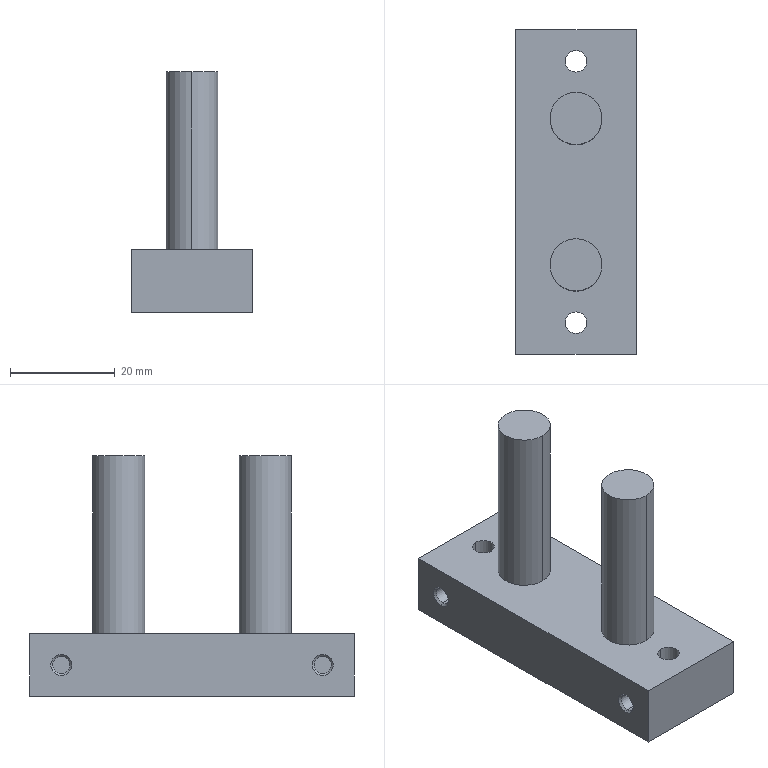Component | SolidWorks | P-SLJ-005-3_CXSM20-20-Z73-1_rod CXSM20-20-Z73-1 | 1 solid | 40 faces | box 23 x 62 x 46 mm | volume 21928 mm3 | cylinder 16 | cone 12 | plane 12 | commonest cylinder face diameters 3.24 x8 4.13 x4 10 x4
STEP:
#1=COLOUR_RGB('',0.7922,0.8196,0.9333);
#2=FILL_AREA_STYLE_COLOUR('',#1);
#3=FILL_AREA_STYLE('',(#2));
#4=SURFACE_STYLE_FILL_AREA(#3);
#5=SURFACE_SIDE_STYLE('',(#4));
#6=SURFACE_STYLE_USAGE(.BOTH.,#5);
#7=PRESENTATION_STYLE_ASSIGNMENT((#6));
#8=CARTESIAN_POINT('',(-2.003,1.594,49.262));
#9=VERTEX_POINT('',#8);
#10=CARTESIAN_POINT('',(-2.003,1.594,49.134));
#11=VERTEX_POINT('',#10);
#12=CARTESIAN_POINT('',(-2.003,1.594,49.198));
#13=DIRECTION('',(-1.,-0.,-0.));
#14=DIRECTION('',(0.,0.,-1.));
#15=AXIS2_PLACEMENT_3D('',#12,#13,#14);
#16=CIRCLE('',#15,0.06378);
#17=EDGE_CURVE('',#9,#11,#16,.T.);
#18=ORIENTED_EDGE('',*,*,#17,.F.);
#19=CARTESIAN_POINT('',(-2.224,1.594,49.262));
#20=VERTEX_POINT('',#19);
#21=CARTESIAN_POINT('',(-1.949,1.594,49.262));
#22=DIRECTION('',(-1.,-0.,-0.));
#23=VECTOR('',#22,39.37);
#24=LINE('',#21,#23);
#25=EDGE_CURVE('',#9,#20,#24,.T.);
#26=ORIENTED_EDGE('',*,*,#25,.T.);
#27=CARTESIAN_POINT('',(-2.224,1.594,49.134));
#28=VERTEX_POINT('',#27);
#29=CARTESIAN_POINT('',(-2.224,1.594,49.198));
#30=DIRECTION('',(-1.,-0.,-0.));
#31=DIRECTION('',(0.,0.,-1.));
#32=AXIS2_PLACEMENT_3D('',#29,#30,#31);
#33=CIRCLE('',#32,0.06378);
#34=EDGE_CURVE('',#20,#28,#33,.T.);
#35=ORIENTED_EDGE('',*,*,#34,.T.);
#36=CARTESIAN_POINT('',(-1.949,1.594,49.134));
#37=DIRECTION('',(-1.,-0.,-0.));
#38=VECTOR('',#37,39.37);
#39=LINE('',#36,#38);
#40=EDGE_CURVE('',#11,#28,#39,.T.);
#41=ORIENTED_EDGE('',*,*,#40,.F.);
#42=EDGE_LOOP('',(#18,#26,#35,#41));
#43=FACE_OUTER_BOUND('',#42,.T.);
#44=CARTESIAN_POINT('',(-1.949,1.594,49.198));
#45=DIRECTION('',(-1.,-0.,-0.));
#46=DIRECTION('',(0.,0.,-1.));
#47=AXIS2_PLACEMENT_3D('',#44,#45,#46);
#48=CYLINDRICAL_SURFACE('',#47,0.06378);
#49=ADVANCED_FACE('',(#43),#48,.F.);
#50=ORIENTED_EDGE('',*,*,#17,.T.);
#51=CARTESIAN_POINT('',(-1.988,1.594,49.119));
#52=VERTEX_POINT('',#51);
#53=CARTESIAN_POINT('',(-1.949,1.594,49.08));
#54=DIRECTION('',(0.7071,0.,-0.7071));
#55=VECTOR('',#54,39.37);
#56=LINE('',#53,#55);
#57=EDGE_CURVE('',#11,#52,#56,.T.);
#58=ORIENTED_EDGE('',*,*,#57,.T.);
#59=CARTESIAN_POINT('',(-1.988,1.594,49.277));
#60=VERTEX_POINT('',#59);
#61=CARTESIAN_POINT('',(-1.988,1.594,49.198));
#62=DIRECTION('',(1.,0.,0.));
#63=DIRECTION('',(0.,0.,-1.));
#64=AXIS2_PLACEMENT_3D('',#61,#62,#63);
#65=CIRCLE('',#64,0.07874);
#66=EDGE_CURVE('',#52,#60,#65,.T.);
#67=ORIENTED_EDGE('',*,*,#66,.T.);
#68=CARTESIAN_POINT('',(-1.949,1.594,49.316));
#69=DIRECTION('',(0.7071,0.,0.7071));
#70=VECTOR('',#69,39.37);
#71=LINE('',#68,#70);
#72=EDGE_CURVE('',#9,#60,#71,.T.);
#73=ORIENTED_EDGE('',*,*,#72,.F.);
#74=EDGE_LOOP('',(#50,#58,#67,#73));
#75=FACE_OUTER_BOUND('',#74,.T.);
#76=CARTESIAN_POINT('',(-1.949,1.594,49.198));
#77=DIRECTION('',(1.,0.,0.));
#78=DIRECTION('',(0.,0.,1.));
#79=AXIS2_PLACEMENT_3D('',#76,#77,#78);
#80=CONICAL_SURFACE('',#79,0.1181,0.7854);
#81=ADVANCED_FACE('',(#75),#80,.F.);
#82=CARTESIAN_POINT('',(-2.003,-0.374,49.262));
#83=VERTEX_POINT('',#82);
#84=CARTESIAN_POINT('',(-2.003,-0.374,49.134));
#85=VERTEX_POINT('',#84);
#86=CARTESIAN_POINT('',(-2.003,-0.374,49.198));
#87=DIRECTION('',(-1.,-0.,-0.));
#88=DIRECTION('',(0.,0.,-1.));
#89=AXIS2_PLACEMENT_3D('',#86,#87,#88);
#90=CIRCLE('',#89,0.06378);
#91=EDGE_CURVE('',#83,#85,#90,.T.);
#92=ORIENTED_EDGE('',*,*,#91,.F.);
#93=CARTESIAN_POINT('',(-2.224,-0.374,49.262));
#94=VERTEX_POINT('',#93);
#95=CARTESIAN_POINT('',(-1.949,-0.374,49.262));
#96=DIRECTION('',(-1.,-0.,-0.));
#97=VECTOR('',#96,39.37);
#98=LINE('',#95,#97);
#99=EDGE_CURVE('',#83,#94,#98,.T.);
#100=ORIENTED_EDGE('',*,*,#99,.T.);
#101=CARTESIAN_POINT('',(-2.224,-0.374,49.134));
#102=VERTEX_POINT('',#101);
#103=CARTESIAN_POINT('',(-2.224,-0.374,49.198));
#104=DIRECTION('',(-1.,-0.,-0.));
#105=DIRECTION('',(0.,0.,-1.));
#106=AXIS2_PLACEMENT_3D('',#103,#104,#105);
#107=CIRCLE('',#106,0.06378);
#108=EDGE_CURVE('',#94,#102,#107,.T.);
#109=ORIENTED_EDGE('',*,*,#108,.T.);
#110=CARTESIAN_POINT('',(-1.949,-0.374,49.134));
#111=DIRECTION('',(-1.,-0.,-0.));
#112=VECTOR('',#111,39.37);
#113=LINE('',#110,#112);
#114=EDGE_CURVE('',#85,#102,#113,.T.);
#115=ORIENTED_EDGE('',*,*,#114,.F.);
#116=EDGE_LOOP('',(#92,#100,#109,#115));
#117=FACE_OUTER_BOUND('',#116,.T.);
#118=CARTESIAN_POINT('',(-1.949,-0.374,49.198));
#119=DIRECTION('',(-1.,-0.,-0.));
#120=DIRECTION('',(0.,0.,-1.));
#121=AXIS2_PLACEMENT_3D('',#118,#119,#120);
#122=CYLINDRICAL_SURFACE('',#121,0.06378);
#123=ADVANCED_FACE('',(#117),#122,.F.);
#124=ORIENTED_EDGE('',*,*,#91,.T.);
#125=CARTESIAN_POINT('',(-1.988,-0.374,49.119));
#126=VERTEX_POINT('',#125);
#127=CARTESIAN_POINT('',(-1.949,-0.374,49.08));
#128=DIRECTION('',(0.7071,0.,-0.7071));
#129=VECTOR('',#128,39.37);
#130=LINE('',#127,#129);
#131=EDGE_CURVE('',#85,#126,#130,.T.);
#132=ORIENTED_EDGE('',*,*,#131,.T.);
#133=CARTESIAN_POINT('',(-1.988,-0.374,49.277));
#134=VERTEX_POINT('',#133);
#135=CARTESIAN_POINT('',(-1.988,-0.374,49.198));
#136=DIRECTION('',(1.,0.,0.));
#137=DIRECTION('',(0.,0.,-1.));
#138=AXIS2_PLACEMENT_3D('',#135,#136,#137);
#139=CIRCLE('',#138,0.07874);
#140=EDGE_CURVE('',#126,#134,#139,.T.);
#141=ORIENTED_EDGE('',*,*,#140,.T.);
#142=CARTESIAN_POINT('',(-1.949,-0.374,49.316));
#143=DIRECTION('',(0.7071,0.,0.7071));
#144=VECTOR('',#143,39.37);
#145=LINE('',#142,#144);
#146=EDGE_CURVE('',#83,#134,#145,.T.);
#147=ORIENTED_EDGE('',*,*,#146,.F.);
#148=EDGE_LOOP('',(#124,#132,#141,#147));
#149=FACE_OUTER_BOUND('',#148,.T.);
#150=CARTESIAN_POINT('',(-1.949,-0.374,49.198));
#151=DIRECTION('',(1.,0.,0.));
#152=DIRECTION('',(0.,0.,1.));
#153=AXIS2_PLACEMENT_3D('',#150,#151,#152);
#154=CONICAL_SURFACE('',#153,0.1181,0.7854);
#155=ADVANCED_FACE('',(#149),#154,.F.);
#156=CARTESIAN_POINT('',(-2.441,1.513,48.979));
#157=VERTEX_POINT('',#156);
#158=CARTESIAN_POINT('',(-2.441,1.676,48.979));
#159=VERTEX_POINT('',#158);
#160=CARTESIAN_POINT('',(-2.441,1.594,48.979));
#161=DIRECTION('',(-0.,0.,1.));
#162=DIRECTION('',(0.,1.,0.));
#163=AXIS2_PLACEMENT_3D('',#160,#161,#162);
#164=CIRCLE('',#163,0.0813);
#165=EDGE_CURVE('',#157,#159,#164,.T.);
#166=ORIENTED_EDGE('',*,*,#165,.T.);
#167=CARTESIAN_POINT('',(-2.441,1.693,48.962));
#168=VERTEX_POINT('',#167);
#169=CARTESIAN_POINT('',(-2.441,1.713,48.942));
#170=DIRECTION('',(-0.,0.7071,-0.7071));
#171=VECTOR('',#170,39.37);
#172=LINE('',#169,#171);
#173=EDGE_CURVE('',#159,#168,#172,.T.);
#174=ORIENTED_EDGE('',*,*,#173,.T.);
#175=CARTESIAN_POINT('',(-2.441,1.496,48.962));
#176=VERTEX_POINT('',#175);
#177=CARTESIAN_POINT('',(-2.441,1.594,48.962));
#178=DIRECTION('',(-0.,0.,1.));
#179=DIRECTION('',(0.,-1.,0.));
#180=AXIS2_PLACEMENT_3D('',#177,#178,#179);
#181=CIRCLE('',#180,0.09843);
#182=EDGE_CURVE('',#176,#168,#181,.T.);
#183=ORIENTED_EDGE('',*,*,#182,.F.);
#184=CARTESIAN_POINT('',(-2.441,1.476,48.942));
#185=DIRECTION('',(0.,-0.7071,-0.7071));
#186=VECTOR('',#185,39.37);
#187=LINE('',#184,#186);
#188=EDGE_CURVE('',#157,#176,#187,.T.);
#189=ORIENTED_EDGE('',*,*,#188,.F.);
#190=EDGE_LOOP('',(#166,#174,#183,#189));
#191=FACE_OUTER_BOUND('',#190,.T.);
#192=CARTESIAN_POINT('',(-2.441,1.594,48.942));
#193=DIRECTION('',(0.,-0.,-1.));
#194=DIRECTION('',(0.,-1.,0.));
#195=AXIS2_PLACEMENT_3D('',#192,#193,#194);
#196=CONICAL_SURFACE('',#195,0.1181,0.7854);
#197=ADVANCED_FACE('',(#191),#196,.F.);
#198=ORIENTED_EDGE('',*,*,#165,.F.);
#199=CARTESIAN_POINT('',(-2.441,1.513,49.434));
#200=VERTEX_POINT('',#199);
#201=CARTESIAN_POINT('',(-2.441,1.513,48.942));
#202=DIRECTION('',(-0.,0.,1.));
#203=VECTOR('',#202,39.37);
#204=LINE('',#201,#203);
#205=EDGE_CURVE('',#157,#200,#204,.T.);
#206=ORIENTED_EDGE('',*,*,#205,.T.);
#207=CARTESIAN_POINT('',(-2.441,1.676,49.434));
#208=VERTEX_POINT('',#207);
#209=CARTESIAN_POINT('',(-2.441,1.594,49.434));
#210=DIRECTION('',(-0.,0.,1.));
#211=DIRECTION('',(0.,1.,0.));
#212=AXIS2_PLACEMENT_3D('',#209,#210,#211);
#213=CIRCLE('',#212,0.0813);
#214=EDGE_CURVE('',#200,#208,#213,.T.);
#215=ORIENTED_EDGE('',*,*,#214,.T.);
#216=CARTESIAN_POINT('',(-2.441,1.676,48.942));
#217=DIRECTION('',(-0.,0.,1.));
#218=VECTOR('',#217,39.37);
#219=LINE('',#216,#218);
#220=EDGE_CURVE('',#159,#208,#219,.T.);
#221=ORIENTED_EDGE('',*,*,#220,.F.);
#222=EDGE_LOOP('',(#198,#206,#215,#221));
#223=FACE_OUTER_BOUND('',#222,.T.);
#224=CARTESIAN_POINT('',(-2.441,1.594,48.942));
#225=DIRECTION('',(-0.,0.,1.));
#226=DIRECTION('',(0.,1.,0.));
#227=AXIS2_PLACEMENT_3D('',#224,#225,#226);
#228=CYLINDRICAL_SURFACE('',#227,0.0813);
#229=ADVANCED_FACE('',(#223),#228,.F.);
#230=CARTESIAN_POINT('',(-2.441,-0.4553,48.979));
#231=VERTEX_POINT('',#230);
#232=CARTESIAN_POINT('',(-2.441,-0.2927,48.979));
#233=VERTEX_POINT('',#232);
#234=CARTESIAN_POINT('',(-2.441,-0.374,48.979));
#235=DIRECTION('',(-0.,0.,1.));
#236=DIRECTION('',(0.,1.,0.));
#237=AXIS2_PLACEMENT_3D('',#234,#235,#236);
#238=CIRCLE('',#237,0.0813);
#239=EDGE_CURVE('',#231,#233,#238,.T.);
#240=ORIENTED_EDGE('',*,*,#239,.T.);
#241=CARTESIAN_POINT('',(-2.441,-0.2756,48.962));
#242=VERTEX_POINT('',#241);
#243=CARTESIAN_POINT('',(-2.441,-0.2559,48.942));
#244=DIRECTION('',(-0.,0.7071,-0.7071));
#245=VECTOR('',#244,39.37);
#246=LINE('',#243,#245);
#247=EDGE_CURVE('',#233,#242,#246,.T.);
#248=ORIENTED_EDGE('',*,*,#247,.T.);
#249=CARTESIAN_POINT('',(-2.441,-0.4724,48.962));
#250=VERTEX_POINT('',#249);
#251=CARTESIAN_POINT('',(-2.441,-0.374,48.962));
#252=DIRECTION('',(-0.,0.,1.));
#253=DIRECTION('',(0.,-1.,0.));
#254=AXIS2_PLACEMENT_3D('',#251,#252,#253);
#255=CIRCLE('',#254,0.09843);
#256=EDGE_CURVE('',#250,#242,#255,.T.);
#257=ORIENTED_EDGE('',*,*,#256,.F.);
#258=CARTESIAN_POINT('',(-2.441,-0.4921,48.942));
#259=DIRECTION('',(0.,-0.7071,-0.7071));
#260=VECTOR('',#259,39.37);
#261=LINE('',#258,#260);
#262=EDGE_CURVE('',#231,#250,#261,.T.);
#263=ORIENTED_EDGE('',*,*,#262,.F.);
#264=EDGE_LOOP('',(#240,#248,#257,#263));
#265=FACE_OUTER_BOUND('',#264,.T.);
#266=CARTESIAN_POINT('',(-2.441,-0.374,48.942));
#267=DIRECTION('',(0.,-0.,-1.));
#268=DIRECTION('',(0.,-1.,0.));
#269=AXIS2_PLACEMENT_3D('',#266,#267,#268);
#270=CONICAL_SURFACE('',#269,0.1181,0.7854);
#271=ADVANCED_FACE('',(#265),#270,.F.);
#272=ORIENTED_EDGE('',*,*,#239,.F.);
#273=CARTESIAN_POINT('',(-2.441,-0.4553,49.434));
#274=VERTEX_POINT('',#273);
#275=CARTESIAN_POINT('',(-2.441,-0.4553,48.942));
#276=DIRECTION('',(-0.,0.,1.));
#277=VECTOR('',#276,39.37);
#278=LINE('',#275,#277);
#279=EDGE_CURVE('',#231,#274,#278,.T.);
#280=ORIENTED_EDGE('',*,*,#279,.T.);
#281=CARTESIAN_POINT('',(-2.441,-0.2927,49.434));
#282=VERTEX_POINT('',#281);
#283=CARTESIAN_POINT('',(-2.441,-0.374,49.434));
#284=DIRECTION('',(-0.,0.,1.));
#285=DIRECTION('',(0.,1.,0.));
#286=AXIS2_PLACEMENT_3D('',#283,#284,#285);
#287=CIRCLE('',#286,0.0813);
#288=EDGE_CURVE('',#274,#282,#287,.T.);
#289=ORIENTED_EDGE('',*,*,#288,.T.);
#290=CARTESIAN_POINT('',(-2.441,-0.2927,48.942));
#291=DIRECTION('',(-0.,0.,1.));
#292=VECTOR('',#291,39.37);
#293=LINE('',#290,#292);
#294=EDGE_CURVE('',#233,#282,#293,.T.);
#295=ORIENTED_EDGE('',*,*,#294,.F.);
#296=EDGE_LOOP('',(#272,#280,#289,#295));
#297=FACE_OUTER_BOUND('',#296,.T.);
#298=CARTESIAN_POINT('',(-2.441,-0.374,48.942));
#299=DIRECTION('',(-0.,0.,1.));
#300=DIRECTION('',(0.,1.,0.));
#301=AXIS2_PLACEMENT_3D('',#298,#299,#300);
#302=CYLINDRICAL_SURFACE('',#301,0.0813);
#303=ADVANCED_FACE('',(#297),#302,.F.);
#304=CARTESIAN_POINT('',(-2.879,-0.374,49.134));
#305=VERTEX_POINT('',#304);
#306=CARTESIAN_POINT('',(-2.879,-0.374,49.262));
#307=VERTEX_POINT('',#306);
#308=CARTESIAN_POINT('',(-2.879,-0.374,49.198));
#309=DIRECTION('',(1.,0.,0.));
#310=DIRECTION('',(0.,0.,1.));
#311=AXIS2_PLACEMENT_3D('',#308,#309,#310);
#312=CIRCLE('',#311,0.06378);
#313=EDGE_CURVE('',#305,#307,#312,.T.);
#314=ORIENTED_EDGE('',*,*,#313,.F.);
#315=CARTESIAN_POINT('',(-2.657,-0.374,49.134));
#316=VERTEX_POINT('',#315);
#317=CARTESIAN_POINT('',(-2.913,-0.374,49.134));
#318=DIRECTION('',(1.,0.,0.));
#319=VECTOR('',#318,39.37);
#320=LINE('',#317,#319);
#321=EDGE_CURVE('',#305,#316,#320,.T.);
#322=ORIENTED_EDGE('',*,*,#321,.T.);
#323=CARTESIAN_POINT('',(-2.657,-0.374,49.262));
#324=VERTEX_POINT('',#323);
#325=CARTESIAN_POINT('',(-2.657,-0.374,49.198));
#326=DIRECTION('',(1.,0.,0.));
#327=DIRECTION('',(0.,0.,1.));
#328=AXIS2_PLACEMENT_3D('',#325,#326,#327);
#329=CIRCLE('',#328,0.06378);
#330=EDGE_CURVE('',#316,#324,#329,.T.);
#331=ORIENTED_EDGE('',*,*,#330,.T.);
#332=CARTESIAN_POINT('',(-2.913,-0.374,49.262));
#333=DIRECTION('',(1.,0.,0.));
#334=VECTOR('',#333,39.37);
#335=LINE('',#332,#334);
#336=EDGE_CURVE('',#307,#324,#335,.T.);
#337=ORIENTED_EDGE('',*,*,#336,.F.);
#338=EDGE_LOOP('',(#314,#322,#331,#337));
#339=FACE_OUTER_BOUND('',#338,.T.);
#340=CARTESIAN_POINT('',(-2.913,-0.374,49.198));
#341=DIRECTION('',(1.,0.,0.));
#342=DIRECTION('',(0.,0.,1.));
#343=AXIS2_PLACEMENT_3D('',#340,#341,#342);
#344=CYLINDRICAL_SURFACE('',#343,0.06378);
#345=ADVANCED_FACE('',(#339),#344,.F.);
#346=ORIENTED_EDGE('',*,*,#313,.T.);
#347=CARTESIAN_POINT('',(-2.894,-0.374,49.277));
#348=VERTEX_POINT('',#347);
#349=CARTESIAN_POINT('',(-2.913,-0.374,49.297));
#350=DIRECTION('',(-0.7071,-0.,0.7071));
#351=VECTOR('',#350,39.37);
#352=LINE('',#349,#351);
#353=EDGE_CURVE('',#307,#348,#352,.T.);
#354=ORIENTED_EDGE('',*,*,#353,.T.);
#355=CARTESIAN_POINT('',(-2.894,-0.374,49.119));
#356=VERTEX_POINT('',#355);
#357=CARTESIAN_POINT('',(-2.894,-0.374,49.198));
#358=DIRECTION('',(-1.,-0.,-0.));
#359=DIRECTION('',(0.,0.,1.));
#360=AXIS2_PLACEMENT_3D('',#357,#358,#359);
#361=CIRCLE('',#360,0.07874);
#362=EDGE_CURVE('',#348,#356,#361,.T.);
#363=ORIENTED_EDGE('',*,*,#362,.T.);
#364=CARTESIAN_POINT('',(-2.913,-0.374,49.1));
#365=DIRECTION('',(-0.7071,-0.,-0.7071));
#366=VECTOR('',#365,39.37);
#367=LINE('',#364,#366);
#368=EDGE_CURVE('',#305,#356,#367,.T.);
#369=ORIENTED_EDGE('',*,*,#368,.F.);
#370=EDGE_LOOP('',(#346,#354,#363,#369));
#371=FACE_OUTER_BOUND('',#370,.T.);
#372=CARTESIAN_POINT('',(-2.913,-0.374,49.198));
#373=DIRECTION('',(-1.,-0.,-0.));
#374=DIRECTION('',(0.,0.,-1.));
#375=AXIS2_PLACEMENT_3D('',#372,#373,#374);
#376=CONICAL_SURFACE('',#375,0.09843,0.7854);
#377=ADVANCED_FACE('',(#371),#376,.F.);
#378=CARTESIAN_POINT('',(-2.879,1.594,49.134));
#379=VERTEX_POINT('',#378);
#380=CARTESIAN_POINT('',(-2.879,1.594,49.262));
#381=VERTEX_POINT('',#380);
#382=CARTESIAN_POINT('',(-2.879,1.594,49.198));
#383=DIRECTION('',(1.,0.,0.));
#384=DIRECTION('',(0.,0.,1.));
#385=AXIS2_PLACEMENT_3D('',#382,#383,#384);
#386=CIRCLE('',#385,0.06378);
#387=EDGE_CURVE('',#379,#381,#386,.T.);
#388=ORIENTED_EDGE('',*,*,#387,.F.);
#389=CARTESIAN_POINT('',(-2.657,1.594,49.134));
#390=VERTEX_POINT('',#389);
#391=CARTESIAN_POINT('',(-2.913,1.594,49.134));
#392=DIRECTION('',(1.,0.,0.));
#393=VECTOR('',#392,39.37);
#394=LINE('',#391,#393);
#395=EDGE_CURVE('',#379,#390,#394,.T.);
#396=ORIENTED_EDGE('',*,*,#395,.T.);
#397=CARTESIAN_POINT('',(-2.657,1.594,49.262));
#398=VERTEX_POINT('',#397);
#399=CARTESIAN_POINT('',(-2.657,1.594,49.198));
#400=DIRECTION('',(1.,0.,0.));
#401=DIRECTION('',(0.,0.,1.));
#402=AXIS2_PLACEMENT_3D('',#399,#400,#401);
#403=CIRCLE('',#402,0.06378);
#404=EDGE_CURVE('',#390,#398,#403,.T.);
#405=ORIENTED_EDGE('',*,*,#404,.T.);
#406=CARTESIAN_POINT('',(-2.913,1.594,49.262));
#407=DIRECTION('',(1.,0.,0.));
#408=VECTOR('',#407,39.37);
#409=LINE('',#406,#408);
#410=EDGE_CURVE('',#381,#398,#409,.T.);
#411=ORIENTED_EDGE('',*,*,#410,.F.);
#412=EDGE_LOOP('',(#388,#396,#405,#411));
#413=FACE_OUTER_BOUND('',#412,.T.);
#414=CARTESIAN_POINT('',(-2.913,1.594,49.198));
#415=DIRECTION('',(1.,0.,0.));
#416=DIRECTION('',(0.,0.,1.));
#417=AXIS2_PLACEMENT_3D('',#414,#415,#416);
#418=CYLINDRICAL_SURFACE('',#417,0.06378);
#419=ADVANCED_FACE('',(#413),#418,.F.);
#420=ORIENTED_EDGE('',*,*,#387,.T.);
#421=CARTESIAN_POINT('',(-2.894,1.594,49.277));
#422=VERTEX_POINT('',#421);
#423=CARTESIAN_POINT('',(-2.913,1.594,49.297));
#424=DIRECTION('',(-0.7071,-0.,0.7071));
#425=VECTOR('',#424,39.37);
#426=LINE('',#423,#425);
#427=EDGE_CURVE('',#381,#422,#426,.T.);
#428=ORIENTED_EDGE('',*,*,#427,.T.);
#429=CARTESIAN_POINT('',(-2.894,1.594,49.119));
#430=VERTEX_POINT('',#429);
#431=CARTESIAN_POINT('',(-2.894,1.594,49.198));
#432=DIRECTION('',(-1.,-0.,-0.));
#433=DIRECTION('',(0.,0.,1.));
#434=AXIS2_PLACEMENT_3D('',#431,#432,#433);
#435=CIRCLE('',#434,0.07874);
#436=EDGE_CURVE('',#422,#430,#435,.T.);
#437=ORIENTED_EDGE('',*,*,#436,.T.);
#438=CARTESIAN_POINT('',(-2.913,1.594,49.1));
#439=DIRECTION('',(-0.7071,-0.,-0.7071));
#440=VECTOR('',#439,39.37);
#441=LINE('',#438,#440);
#442=EDGE_CURVE('',#379,#430,#441,.T.);
#443=ORIENTED_EDGE('',*,*,#442,.F.);
#444=EDGE_LOOP('',(#420,#428,#437,#443));
#445=FACE_OUTER_BOUND('',#444,.T.);
#446=CARTESIAN_POINT('',(-2.913,1.594,49.198));
#447=DIRECTION('',(-1.,-0.,-0.));
#448=DIRECTION('',(0.,0.,-1.));
#449=AXIS2_PLACEMENT_3D('',#446,#447,#448);
#450=CONICAL_SURFACE('',#449,0.09843,0.7854);
#451=ADVANCED_FACE('',(#445),#450,.F.);
#452=CARTESIAN_POINT('',(-2.441,0.9646,50.773));
#453=VERTEX_POINT('',#452);
#454=CARTESIAN_POINT('',(-2.441,1.358,50.773));
#455=VERTEX_POINT('',#454);
#456=CARTESIAN_POINT('',(-2.441,1.161,50.773));
#457=DIRECTION('',(0.,-0.,-1.));
#458=DIRECTION('',(0.,-1.,0.));
#459=AXIS2_PLACEMENT_3D('',#456,#457,#458);
#460=CIRCLE('',#459,0.1969);
#461=EDGE_CURVE('',#453,#455,#460,.T.);
#462=ORIENTED_EDGE('',*,*,#461,.T.);
#463=CARTESIAN_POINT('',(-2.441,1.358,49.434));
#464=VERTEX_POINT('',#463);
#465=CARTESIAN_POINT('',(-2.441,1.358,50.773));
#466=DIRECTION('',(0.,-0.,-1.));
#467=VECTOR('',#466,39.37);
#468=LINE('',#465,#467);
#469=EDGE_CURVE('',#455,#464,#468,.T.);
#470=ORIENTED_EDGE('',*,*,#469,.T.);
#471=CARTESIAN_POINT('',(-2.441,0.9646,49.434));
#472=VERTEX_POINT('',#471);
#473=CARTESIAN_POINT('',(-2.441,1.161,49.434));
#474=DIRECTION('',(0.,-0.,-1.));
#475=DIRECTION('',(0.,-1.,0.));
#476=AXIS2_PLACEMENT_3D('',#473,#474,#475);
#477=CIRCLE('',#476,0.1969);
#478=EDGE_CURVE('',#472,#464,#477,.T.);
#479=ORIENTED_EDGE('',*,*,#478,.F.);
#480=CARTESIAN_POINT('',(-2.441,0.9646,50.773));
#481=DIRECTION('',(0.,-0.,-1.));
#482=VECTOR('',#481,39.37);
#483=LINE('',#480,#482);
#484=EDGE_CURVE('',#453,#472,#483,.T.);
#485=ORIENTED_EDGE('',*,*,#484,.F.);
#486=EDGE_LOOP('',(#462,#470,#479,#485));
#487=FACE_OUTER_BOUND('',#486,.T.);
#488=CARTESIAN_POINT('',(-2.441,1.161,50.773));
#489=DIRECTION('',(0.,-0.,-1.));
#490=DIRECTION('',(0.,-1.,0.));
#491=AXIS2_PLACEMENT_3D('',#488,#489,#490);
#492=CYLINDRICAL_SURFACE('',#491,0.1969);
#493=ADVANCED_FACE('',(#487),#492,.T.);
#494=CARTESIAN_POINT('',(-2.441,-0.1378,50.773));
#495=VERTEX_POINT('',#494);
#496=CARTESIAN_POINT('',(-2.441,0.2559,50.773));
#497=VERTEX_POINT('',#496);
#498=CARTESIAN_POINT('',(-2.441,0.05906,50.773));
#499=DIRECTION('',(0.,-0.,-1.));
#500=DIRECTION('',(0.,-1.,0.));
#501=AXIS2_PLACEMENT_3D('',#498,#499,#500);
#502=CIRCLE('',#501,0.1969);
#503=EDGE_CURVE('',#495,#497,#502,.T.);
#504=ORIENTED_EDGE('',*,*,#503,.T.);
#505=CARTESIAN_POINT('',(-2.441,0.2559,49.434));
#506=VERTEX_POINT('',#505);
#507=CARTESIAN_POINT('',(-2.441,0.2559,50.773));
#508=DIRECTION('',(0.,-0.,-1.));
#509=VECTOR('',#508,39.37);
#510=LINE('',#507,#509);
#511=EDGE_CURVE('',#497,#506,#510,.T.);
#512=ORIENTED_EDGE('',*,*,#511,.T.);
#513=CARTESIAN_POINT('',(-2.441,-0.1378,49.434));
#514=VERTEX_POINT('',#513);
#515=CARTESIAN_POINT('',(-2.441,0.05906,49.434));
#516=DIRECTION('',(0.,-0.,-1.));
#517=DIRECTION('',(0.,-1.,0.));
#518=AXIS2_PLACEMENT_3D('',#515,#516,#517);
#519=CIRCLE('',#518,0.1969);
#520=EDGE_CURVE('',#514,#506,#519,.T.);
#521=ORIENTED_EDGE('',*,*,#520,.F.);
#522=CARTESIAN_POINT('',(-2.441,-0.1378,50.773));
#523=DIRECTION('',(0.,-0.,-1.));
#524=VECTOR('',#523,39.37);
#525=LINE('',#522,#524);
#526=EDGE_CURVE('',#495,#514,#525,.T.);
#527=ORIENTED_EDGE('',*,*,#526,.F.);
#528=EDGE_LOOP('',(#504,#512,#521,#527));
#529=FACE_OUTER_BOUND('',#528,.T.);
#530=CARTESIAN_POINT('',(-2.441,0.05906,50.773));
#531=DIRECTION('',(0.,-0.,-1.));
#532=DIRECTION('',(0.,-1.,0.));
#533=AXIS2_PLACEMENT_3D('',#530,#531,#532);
#534=CYLINDRICAL_SURFACE('',#533,0.1969);
#535=ADVANCED_FACE('',(#529),#534,.T.);
#536=CARTESIAN_POINT('',(-1.988,-0.374,49.198));
#537=DIRECTION('',(1.,0.,0.));
#538=DIRECTION('',(0.,0.,-1.));
#539=AXIS2_PLACEMENT_3D('',#536,#537,#538);
#540=CIRCLE('',#539,0.07874);
#541=EDGE_CURVE('',#134,#126,#540,.T.);
#542=ORIENTED_EDGE('',*,*,#541,.F.);
#543=ORIENTED_EDGE('',*,*,#140,.F.);
#544=EDGE_LOOP('',(#542,#543));
#545=FACE_BOUND('',#544,.T.);
#546=CARTESIAN_POINT('',(-1.988,1.831,49.434));
#547=VERTEX_POINT('',#546);
#548=CARTESIAN_POINT('',(-1.988,-0.6102,49.434));
#549=VERTEX_POINT('',#548);
#550=CARTESIAN_POINT('',(-1.988,1.831,49.434));
#551=DIRECTION('',(0.,-1.,-0.));
#552=VECTOR('',#551,39.37);
#553=LINE('',#550,#552);
#554=EDGE_CURVE('',#547,#549,#553,.T.);
#555=ORIENTED_EDGE('',*,*,#554,.T.);
#556=CARTESIAN_POINT('',(-1.988,-0.6102,48.962));
#557=VERTEX_POINT('',#556);
#558=CARTESIAN_POINT('',(-1.988,-0.6102,48.962));
#559=DIRECTION('',(-0.,0.,1.));
#560=VECTOR('',#559,39.37);
#561=LINE('',#558,#560);
#562=EDGE_CURVE('',#557,#549,#561,.T.);
#563=ORIENTED_EDGE('',*,*,#562,.F.);
#564=CARTESIAN_POINT('',(-1.988,1.831,48.962));
#565=VERTEX_POINT('',#564);
#566=CARTESIAN_POINT('',(-1.988,1.831,48.962));
#567=DIRECTION('',(0.,-1.,-0.));
#568=VECTOR('',#567,39.37);
#569=LINE('',#566,#568);
#570=EDGE_CURVE('',#565,#557,#569,.T.);
#571=ORIENTED_EDGE('',*,*,#570,.F.);
#572=CARTESIAN_POINT('',(-1.988,1.831,48.962));
#573=DIRECTION('',(-0.,0.,1.));
#574=VECTOR('',#573,39.37);
#575=LINE('',#572,#574);
#576=EDGE_CURVE('',#565,#547,#575,.T.);
#577=ORIENTED_EDGE('',*,*,#576,.T.);
#578=EDGE_LOOP('',(#555,#563,#571,#577));
#579=FACE_OUTER_BOUND('',#578,.T.);
#580=CARTESIAN_POINT('',(-1.988,1.594,49.198));
#581=DIRECTION('',(1.,0.,0.));
#582=DIRECTION('',(0.,0.,-1.));
#583=AXIS2_PLACEMENT_3D('',#580,#581,#582);
#584=CIRCLE('',#583,0.07874);
#585=EDGE_CURVE('',#60,#52,#584,.T.);
#586=ORIENTED_EDGE('',*,*,#585,.F.);
#587=ORIENTED_EDGE('',*,*,#66,.F.);
#588=EDGE_LOOP('',(#586,#587));
#589=FACE_BOUND('',#588,.T.);
#590=CARTESIAN_POINT('',(-1.988,1.831,48.962));
#591=DIRECTION('',(-1.,-0.,-0.));
#592=DIRECTION('',(0.,-0.,-1.));
#593=AXIS2_PLACEMENT_3D('',#590,#591,#592);
#594=PLANE('',#593);
#595=ADVANCED_FACE('',(#545,#579,#589),#594,.F.);
#596=ORIENTED_EDGE('',*,*,#256,.T.);
#597=CARTESIAN_POINT('',(-2.441,-0.374,48.962));
#598=DIRECTION('',(-0.,0.,1.));
#599=DIRECTION('',(0.,-1.,0.));
#600=AXIS2_PLACEMENT_3D('',#597,#598,#599);
#601=CIRCLE('',#600,0.09843);
#602=EDGE_CURVE('',#242,#250,#601,.T.);
#603=ORIENTED_EDGE('',*,*,#602,.T.);
#604=EDGE_LOOP('',(#596,#603));
#605=FACE_BOUND('',#604,.T.);
#606=CARTESIAN_POINT('',(-2.894,1.831,48.962));
#607=VERTEX_POINT('',#606);
#608=CARTESIAN_POINT('',(-2.894,1.831,48.962));
#609=DIRECTION('',(1.,0.,0.));
#610=VECTOR('',#609,39.37);
#611=LINE('',#608,#610);
#612=EDGE_CURVE('',#607,#565,#611,.T.);
#613=ORIENTED_EDGE('',*,*,#612,.T.);
#614=ORIENTED_EDGE('',*,*,#570,.T.);
#615=CARTESIAN_POINT('',(-2.894,-0.6102,48.962));
#616=VERTEX_POINT('',#615);
#617=CARTESIAN_POINT('',(-1.988,-0.6102,48.962));
#618=DIRECTION('',(-1.,-0.,-0.));
#619=VECTOR('',#618,39.37);
#620=LINE('',#617,#619);
#621=EDGE_CURVE('',#557,#616,#620,.T.);
#622=ORIENTED_EDGE('',*,*,#621,.T.);
#623=CARTESIAN_POINT('',(-2.894,-0.6102,48.962));
#624=DIRECTION('',(-0.,1.,0.));
#625=VECTOR('',#624,39.37);
#626=LINE('',#623,#625);
#627=EDGE_CURVE('',#616,#607,#626,.T.);
#628=ORIENTED_EDGE('',*,*,#627,.T.);
#629=EDGE_LOOP('',(#613,#614,#622,#628));
#630=FACE_OUTER_BOUND('',#629,.T.);
#631=ORIENTED_EDGE('',*,*,#182,.T.);
#632=CARTESIAN_POINT('',(-2.441,1.594,48.962));
#633=DIRECTION('',(-0.,0.,1.));
#634=DIRECTION('',(0.,-1.,0.));
#635=AXIS2_PLACEMENT_3D('',#632,#633,#634);
#636=CIRCLE('',#635,0.09843);
#637=EDGE_CURVE('',#168,#176,#636,.T.);
#638=ORIENTED_EDGE('',*,*,#637,.T.);
#639=EDGE_LOOP('',(#631,#638));
#640=FACE_BOUND('',#639,.T.);
#641=CARTESIAN_POINT('',(-1.949,0.6102,48.962));
#642=DIRECTION('',(0.,0.,-1.));
#643=DIRECTION('',(0.,-1.,-0.));
#644=AXIS2_PLACEMENT_3D('',#641,#642,#643);
#645=PLANE('',#644);
#646=ADVANCED_FACE('',(#605,#630,#640),#645,.T.);
#647=CARTESIAN_POINT('',(-2.441,-0.374,49.434));
#648=DIRECTION('',(-0.,0.,1.));
#649=DIRECTION('',(0.,1.,0.));
#650=AXIS2_PLACEMENT_3D('',#647,#648,#649);
#651=CIRCLE('',#650,0.0813);
#652=EDGE_CURVE('',#282,#274,#651,.T.);
#653=ORIENTED_EDGE('',*,*,#652,.F.);
#654=ORIENTED_EDGE('',*,*,#288,.F.);
#655=EDGE_LOOP('',(#653,#654));
#656=FACE_BOUND('',#655,.T.);
#657=ORIENTED_EDGE('',*,*,#478,.T.);
#658=CARTESIAN_POINT('',(-2.441,1.161,49.434));
#659=DIRECTION('',(0.,-0.,-1.));
#660=DIRECTION('',(0.,-1.,0.));
#661=AXIS2_PLACEMENT_3D('',#658,#659,#660);
#662=CIRCLE('',#661,0.1969);
#663=EDGE_CURVE('',#464,#472,#662,.T.);
#664=ORIENTED_EDGE('',*,*,#663,.T.);
#665=EDGE_LOOP('',(#657,#664));
#666=FACE_BOUND('',#665,.T.);
#667=ORIENTED_EDGE('',*,*,#520,.T.);
#668=CARTESIAN_POINT('',(-2.441,0.05906,49.434));
#669=DIRECTION('',(0.,-0.,-1.));
#670=DIRECTION('',(0.,-1.,0.));
#671=AXIS2_PLACEMENT_3D('',#668,#669,#670);
#672=CIRCLE('',#671,0.1969);
#673=EDGE_CURVE('',#506,#514,#672,.T.);
#674=ORIENTED_EDGE('',*,*,#673,.T.);
#675=EDGE_LOOP('',(#667,#674));
#676=FACE_BOUND('',#675,.T.);
#677=CARTESIAN_POINT('',(-2.894,1.831,49.434));
#678=VERTEX_POINT('',#677);
#679=CARTESIAN_POINT('',(-2.894,1.831,49.434));
#680=DIRECTION('',(1.,0.,0.));
#681=VECTOR('',#680,39.37);
#682=LINE('',#679,#681);
#683=EDGE_CURVE('',#678,#547,#682,.T.);
#684=ORIENTED_EDGE('',*,*,#683,.F.);
#685=CARTESIAN_POINT('',(-2.894,-0.6102,49.434));
#686=VERTEX_POINT('',#685);
#687=CARTESIAN_POINT('',(-2.894,-0.6102,49.434));
#688=DIRECTION('',(-0.,1.,0.));
#689=VECTOR('',#688,39.37);
#690=LINE('',#687,#689);
#691=EDGE_CURVE('',#686,#678,#690,.T.);
#692=ORIENTED_EDGE('',*,*,#691,.F.);
#693=CARTESIAN_POINT('',(-1.988,-0.6102,49.434));
#694=DIRECTION('',(-1.,-0.,-0.));
#695=VECTOR('',#694,39.37);
#696=LINE('',#693,#695);
#697=EDGE_CURVE('',#549,#686,#696,.T.);
#698=ORIENTED_EDGE('',*,*,#697,.F.);
#699=ORIENTED_EDGE('',*,*,#554,.F.);
#700=EDGE_LOOP('',(#684,#692,#698,#699));
#701=FACE_OUTER_BOUND('',#700,.T.);
#702=CARTESIAN_POINT('',(-2.441,1.594,49.434));
#703=DIRECTION('',(-0.,0.,1.));
#704=DIRECTION('',(0.,1.,0.));
#705=AXIS2_PLACEMENT_3D('',#702,#703,#704);
#706=CIRCLE('',#705,0.0813);
#707=EDGE_CURVE('',#208,#200,#706,.T.);
#708=ORIENTED_EDGE('',*,*,#707,.F.);
#709=ORIENTED_EDGE('',*,*,#214,.F.);
#710=EDGE_LOOP('',(#708,#709));
#711=FACE_BOUND('',#710,.T.);
#712=CARTESIAN_POINT('',(-1.949,0.6102,49.434));
#713=DIRECTION('',(0.,0.,-1.));
#714=DIRECTION('',(0.,-1.,-0.));
#715=AXIS2_PLACEMENT_3D('',#712,#713,#714);
#716=PLANE('',#715);
#717=ADVANCED_FACE('',(#656,#666,#676,#701,#711),#716,.F.);
#718=CARTESIAN_POINT('',(-2.894,1.594,49.198));
#719=DIRECTION('',(-1.,-0.,-0.));
#720=DIRECTION('',(0.,0.,1.));
#721=AXIS2_PLACEMENT_3D('',#718,#719,#720);
#722=CIRCLE('',#721,0.07874);
#723=EDGE_CURVE('',#430,#422,#722,.T.);
#724=ORIENTED_EDGE('',*,*,#723,.F.);
#725=ORIENTED_EDGE('',*,*,#436,.F.);
#726=EDGE_LOOP('',(#724,#725));
#727=FACE_BOUND('',#726,.T.);
#728=ORIENTED_EDGE('',*,*,#691,.T.);
#729=CARTESIAN_POINT('',(-2.894,1.831,48.962));
#730=DIRECTION('',(-0.,0.,1.));
#731=VECTOR('',#730,39.37);
#732=LINE('',#729,#731);
#733=EDGE_CURVE('',#607,#678,#732,.T.);
#734=ORIENTED_EDGE('',*,*,#733,.F.);
#735=ORIENTED_EDGE('',*,*,#627,.F.);
#736=CARTESIAN_POINT('',(-2.894,-0.6102,48.962));
#737=DIRECTION('',(-0.,0.,1.));
#738=VECTOR('',#737,39.37);
#739=LINE('',#736,#738);
#740=EDGE_CURVE('',#616,#686,#739,.T.);
#741=ORIENTED_EDGE('',*,*,#740,.T.);
#742=EDGE_LOOP('',(#728,#734,#735,#741));
#743=FACE_OUTER_BOUND('',#742,.T.);
#744=CARTESIAN_POINT('',(-2.894,-0.374,49.198));
#745=DIRECTION('',(-1.,-0.,-0.));
#746=DIRECTION('',(0.,0.,1.));
#747=AXIS2_PLACEMENT_3D('',#744,#745,#746);
#748=CIRCLE('',#747,0.07874);
#749=EDGE_CURVE('',#356,#348,#748,.T.);
#750=ORIENTED_EDGE('',*,*,#749,.F.);
#751=ORIENTED_EDGE('',*,*,#362,.F.);
#752=EDGE_LOOP('',(#750,#751));
#753=FACE_BOUND('',#752,.T.);
#754=CARTESIAN_POINT('',(-2.894,-0.6102,48.962));
#755=DIRECTION('',(1.,0.,0.));
#756=DIRECTION('',(-0.,0.,1.));
#757=AXIS2_PLACEMENT_3D('',#754,#755,#756);
#758=PLANE('',#757);
#759=ADVANCED_FACE('',(#727,#743,#753),#758,.F.);
#760=ORIENTED_EDGE('',*,*,#683,.T.);
#761=ORIENTED_EDGE('',*,*,#576,.F.);
#762=ORIENTED_EDGE('',*,*,#612,.F.);
#763=ORIENTED_EDGE('',*,*,#733,.T.);
#764=EDGE_LOOP('',(#760,#761,#762,#763));
#765=FACE_OUTER_BOUND('',#764,.T.);
#766=CARTESIAN_POINT('',(-2.894,1.831,48.962));
#767=DIRECTION('',(0.,-1.,0.));
#768=DIRECTION('',(-0.,0.,1.));
#769=AXIS2_PLACEMENT_3D('',#766,#767,#768);
#770=PLANE('',#769);
#771=ADVANCED_FACE('',(#765),#770,.F.);
#772=ORIENTED_EDGE('',*,*,#697,.T.);
#773=ORIENTED_EDGE('',*,*,#740,.F.);
#774=ORIENTED_EDGE('',*,*,#621,.F.);
#775=ORIENTED_EDGE('',*,*,#562,.T.);
#776=EDGE_LOOP('',(#772,#773,#774,#775));
#777=FACE_OUTER_BOUND('',#776,.T.);
#778=CARTESIAN_POINT('',(-1.988,-0.6102,48.962));
#779=DIRECTION('',(-0.,1.,-0.));
#780=DIRECTION('',(0.,-0.,-1.));
#781=AXIS2_PLACEMENT_3D('',#778,#779,#780);
#782=PLANE('',#781);
#783=ADVANCED_FACE('',(#777),#782,.F.);
#784=ORIENTED_EDGE('',*,*,#511,.F.);
#785=CARTESIAN_POINT('',(-2.441,0.05906,50.773));
#786=DIRECTION('',(0.,-0.,-1.));
#787=DIRECTION('',(0.,-1.,0.));
#788=AXIS2_PLACEMENT_3D('',#785,#786,#787);
#789=CIRCLE('',#788,0.1969);
#790=EDGE_CURVE('',#497,#495,#789,.T.);
#791=ORIENTED_EDGE('',*,*,#790,.T.);
#792=ORIENTED_EDGE('',*,*,#526,.T.);
#793=ORIENTED_EDGE('',*,*,#673,.F.);
#794=EDGE_LOOP('',(#784,#791,#792,#793));
#795=FACE_OUTER_BOUND('',#794,.T.);
#796=CARTESIAN_POINT('',(-2.441,0.05906,50.773));
#797=DIRECTION('',(0.,-0.,-1.));
#798=DIRECTION('',(0.,-1.,0.));
#799=AXIS2_PLACEMENT_3D('',#796,#797,#798);
#800=CYLINDRICAL_SURFACE('',#799,0.1969);
#801=ADVANCED_FACE('',(#795),#800,.T.);
#802=ORIENTED_EDGE('',*,*,#503,.F.);
#803=ORIENTED_EDGE('',*,*,#790,.F.);
#804=EDGE_LOOP('',(#802,#803));
#805=FACE_OUTER_BOUND('',#804,.T.);
#806=CARTESIAN_POINT('',(-2.441,0.05906,50.773));
#807=DIRECTION('',(0.,0.,-1.));
#808=DIRECTION('',(0.,-1.,-0.));
#809=AXIS2_PLACEMENT_3D('',#806,#807,#808);
#810=PLANE('',#809);
#811=ADVANCED_FACE('',(#805),#810,.F.);
#812=ORIENTED_EDGE('',*,*,#469,.F.);
#813=CARTESIAN_POINT('',(-2.441,1.161,50.773));
#814=DIRECTION('',(0.,-0.,-1.));
#815=DIRECTION('',(0.,-1.,0.));
#816=AXIS2_PLACEMENT_3D('',#813,#814,#815);
#817=CIRCLE('',#816,0.1969);
#818=EDGE_CURVE('',#455,#453,#817,.T.);
#819=ORIENTED_EDGE('',*,*,#818,.T.);
#820=ORIENTED_EDGE('',*,*,#484,.T.);
#821=ORIENTED_EDGE('',*,*,#663,.F.);
#822=EDGE_LOOP('',(#812,#819,#820,#821));
#823=FACE_OUTER_BOUND('',#822,.T.);
#824=CARTESIAN_POINT('',(-2.441,1.161,50.773));
#825=DIRECTION('',(0.,-0.,-1.));
#826=DIRECTION('',(0.,-1.,0.));
#827=AXIS2_PLACEMENT_3D('',#824,#825,#826);
#828=CYLINDRICAL_SURFACE('',#827,0.1969);
#829=ADVANCED_FACE('',(#823),#828,.T.);
#830=ORIENTED_EDGE('',*,*,#461,.F.);
#831=ORIENTED_EDGE('',*,*,#818,.F.);
#832=EDGE_LOOP('',(#830,#831));
#833=FACE_OUTER_BOUND('',#832,.T.);
#834=CARTESIAN_POINT('',(-2.441,1.161,50.773));
#835=DIRECTION('',(0.,0.,-1.));
#836=DIRECTION('',(0.,-1.,-0.));
#837=AXIS2_PLACEMENT_3D('',#834,#835,#836);
#838=PLANE('',#837);
#839=ADVANCED_FACE('',(#833),#838,.F.);
#840=ORIENTED_EDGE('',*,*,#427,.F.);
#841=CARTESIAN_POINT('',(-2.879,1.594,49.198));
#842=DIRECTION('',(1.,0.,0.));
#843=DIRECTION('',(0.,0.,1.));
#844=AXIS2_PLACEMENT_3D('',#841,#842,#843);
#845=CIRCLE('',#844,0.06378);
#846=EDGE_CURVE('',#381,#379,#845,.T.);
#847=ORIENTED_EDGE('',*,*,#846,.T.);
#848=ORIENTED_EDGE('',*,*,#442,.T.);
#849=ORIENTED_EDGE('',*,*,#723,.T.);
#850=EDGE_LOOP('',(#840,#847,#848,#849));
#851=FACE_OUTER_BOUND('',#850,.T.);
#852=CARTESIAN_POINT('',(-2.913,1.594,49.198));
#853=DIRECTION('',(-1.,-0.,-0.));
#854=DIRECTION('',(0.,0.,-1.));
#855=AXIS2_PLACEMENT_3D('',#852,#853,#854);
#856=CONICAL_SURFACE('',#855,0.09843,0.7854);
#857=ADVANCED_FACE('',(#851),#856,.F.);
#858=CARTESIAN_POINT('',(-2.657,1.594,49.198));
#859=DIRECTION('',(1.,0.,0.));
#860=DIRECTION('',(0.,0.,1.));
#861=AXIS2_PLACEMENT_3D('',#858,#859,#860);
#862=CIRCLE('',#861,0.06378);
#863=EDGE_CURVE('',#398,#390,#862,.T.);
#864=ORIENTED_EDGE('',*,*,#863,.F.);
#865=ORIENTED_EDGE('',*,*,#404,.F.);
#866=EDGE_LOOP('',(#864,#865));
#867=FACE_OUTER_BOUND('',#866,.T.);
#868=CARTESIAN_POINT('',(-2.657,1.594,49.198));
#869=DIRECTION('',(-1.,-0.,-0.));
#870=DIRECTION('',(0.,-0.,-1.));
#871=AXIS2_PLACEMENT_3D('',#868,#869,#870);
#872=PLANE('',#871);
#873=ADVANCED_FACE('',(#867),#872,.T.);
#874=ORIENTED_EDGE('',*,*,#395,.F.);
#875=ORIENTED_EDGE('',*,*,#846,.F.);
#876=ORIENTED_EDGE('',*,*,#410,.T.);
#877=ORIENTED_EDGE('',*,*,#863,.T.);
#878=EDGE_LOOP('',(#874,#875,#876,#877));
#879=FACE_OUTER_BOUND('',#878,.T.);
#880=CARTESIAN_POINT('',(-2.913,1.594,49.198));
#881=DIRECTION('',(1.,0.,0.));
#882=DIRECTION('',(0.,0.,1.));
#883=AXIS2_PLACEMENT_3D('',#880,#881,#882);
#884=CYLINDRICAL_SURFACE('',#883,0.06378);
#885=ADVANCED_FACE('',(#879),#884,.F.);
#886=ORIENTED_EDGE('',*,*,#353,.F.);
#887=CARTESIAN_POINT('',(-2.879,-0.374,49.198));
#888=DIRECTION('',(1.,0.,0.));
#889=DIRECTION('',(0.,0.,1.));
#890=AXIS2_PLACEMENT_3D('',#887,#888,#889);
#891=CIRCLE('',#890,0.06378);
#892=EDGE_CURVE('',#307,#305,#891,.T.);
#893=ORIENTED_EDGE('',*,*,#892,.T.);
#894=ORIENTED_EDGE('',*,*,#368,.T.);
#895=ORIENTED_EDGE('',*,*,#749,.T.);
#896=EDGE_LOOP('',(#886,#893,#894,#895));
#897=FACE_OUTER_BOUND('',#896,.T.);
#898=CARTESIAN_POINT('',(-2.913,-0.374,49.198));
#899=DIRECTION('',(-1.,-0.,-0.));
#900=DIRECTION('',(0.,0.,-1.));
#901=AXIS2_PLACEMENT_3D('',#898,#899,#900);
#902=CONICAL_SURFACE('',#901,0.09843,0.7854);
#903=ADVANCED_FACE('',(#897),#902,.F.);
#904=CARTESIAN_POINT('',(-2.657,-0.374,49.198));
#905=DIRECTION('',(1.,0.,0.));
#906=DIRECTION('',(0.,0.,1.));
#907=AXIS2_PLACEMENT_3D('',#904,#905,#906);
#908=CIRCLE('',#907,0.06378);
#909=EDGE_CURVE('',#324,#316,#908,.T.);
#910=ORIENTED_EDGE('',*,*,#909,.F.);
#911=ORIENTED_EDGE('',*,*,#330,.F.);
#912=EDGE_LOOP('',(#910,#911));
#913=FACE_OUTER_BOUND('',#912,.T.);
#914=CARTESIAN_POINT('',(-2.657,-0.374,49.198));
#915=DIRECTION('',(-1.,-0.,-0.));
#916=DIRECTION('',(0.,-0.,-1.));
#917=AXIS2_PLACEMENT_3D('',#914,#915,#916);
#918=PLANE('',#917);
#919=ADVANCED_FACE('',(#913),#918,.T.);
#920=ORIENTED_EDGE('',*,*,#321,.F.);
#921=ORIENTED_EDGE('',*,*,#892,.F.);
#922=ORIENTED_EDGE('',*,*,#336,.T.);
#923=ORIENTED_EDGE('',*,*,#909,.T.);
#924=EDGE_LOOP('',(#920,#921,#922,#923));
#925=FACE_OUTER_BOUND('',#924,.T.);
#926=CARTESIAN_POINT('',(-2.913,-0.374,49.198));
#927=DIRECTION('',(1.,0.,0.));
#928=DIRECTION('',(0.,0.,1.));
#929=AXIS2_PLACEMENT_3D('',#926,#927,#928);
#930=CYLINDRICAL_SURFACE('',#929,0.06378);
#931=ADVANCED_FACE('',(#925),#930,.F.);
#932=ORIENTED_EDGE('',*,*,#279,.F.);
#933=CARTESIAN_POINT('',(-2.441,-0.374,48.979));
#934=DIRECTION('',(-0.,0.,1.));
#935=DIRECTION('',(0.,1.,0.));
#936=AXIS2_PLACEMENT_3D('',#933,#934,#935);
#937=CIRCLE('',#936,0.0813);
#938=EDGE_CURVE('',#233,#231,#937,.T.);
#939=ORIENTED_EDGE('',*,*,#938,.F.);
#940=ORIENTED_EDGE('',*,*,#294,.T.);
#941=ORIENTED_EDGE('',*,*,#652,.T.);
#942=EDGE_LOOP('',(#932,#939,#940,#941));
#943=FACE_OUTER_BOUND('',#942,.T.);
#944=CARTESIAN_POINT('',(-2.441,-0.374,48.942));
#945=DIRECTION('',(-0.,0.,1.));
#946=DIRECTION('',(0.,1.,0.));
#947=AXIS2_PLACEMENT_3D('',#944,#945,#946);
#948=CYLINDRICAL_SURFACE('',#947,0.0813);
#949=ADVANCED_FACE('',(#943),#948,.F.);
#950=ORIENTED_EDGE('',*,*,#247,.F.);
#951=ORIENTED_EDGE('',*,*,#938,.T.);
#952=ORIENTED_EDGE('',*,*,#262,.T.);
#953=ORIENTED_EDGE('',*,*,#602,.F.);
#954=EDGE_LOOP('',(#950,#951,#952,#953));
#955=FACE_OUTER_BOUND('',#954,.T.);
#956=CARTESIAN_POINT('',(-2.441,-0.374,48.942));
#957=DIRECTION('',(0.,-0.,-1.));
#958=DIRECTION('',(0.,-1.,0.));
#959=AXIS2_PLACEMENT_3D('',#956,#957,#958);
#960=CONICAL_SURFACE('',#959,0.1181,0.7854);
#961=ADVANCED_FACE('',(#955),#960,.F.);
#962=ORIENTED_EDGE('',*,*,#205,.F.);
#963=CARTESIAN_POINT('',(-2.441,1.594,48.979));
#964=DIRECTION('',(-0.,0.,1.));
#965=DIRECTION('',(0.,1.,0.));
#966=AXIS2_PLACEMENT_3D('',#963,#964,#965);
#967=CIRCLE('',#966,0.0813);
#968=EDGE_CURVE('',#159,#157,#967,.T.);
#969=ORIENTED_EDGE('',*,*,#968,.F.);
#970=ORIENTED_EDGE('',*,*,#220,.T.);
#971=ORIENTED_EDGE('',*,*,#707,.T.);
#972=EDGE_LOOP('',(#962,#969,#970,#971));
#973=FACE_OUTER_BOUND('',#972,.T.);
#974=CARTESIAN_POINT('',(-2.441,1.594,48.942));
#975=DIRECTION('',(-0.,0.,1.));
#976=DIRECTION('',(0.,1.,0.));
#977=AXIS2_PLACEMENT_3D('',#974,#975,#976);
#978=CYLINDRICAL_SURFACE('',#977,0.0813);
#979=ADVANCED_FACE('',(#973),#978,.F.);
#980=ORIENTED_EDGE('',*,*,#173,.F.);
#981=ORIENTED_EDGE('',*,*,#968,.T.);
#982=ORIENTED_EDGE('',*,*,#188,.T.);
#983=ORIENTED_EDGE('',*,*,#637,.F.);
#984=EDGE_LOOP('',(#980,#981,#982,#983));
#985=FACE_OUTER_BOUND('',#984,.T.);
#986=CARTESIAN_POINT('',(-2.441,1.594,48.942));
#987=DIRECTION('',(0.,-0.,-1.));
#988=DIRECTION('',(0.,-1.,0.));
#989=AXIS2_PLACEMENT_3D('',#986,#987,#988);
#990=CONICAL_SURFACE('',#989,0.1181,0.7854);
#991=ADVANCED_FACE('',(#985),#990,.F.);
#992=ORIENTED_EDGE('',*,*,#131,.F.);
#993=CARTESIAN_POINT('',(-2.003,-0.374,49.198));
#994=DIRECTION('',(-1.,-0.,-0.));
#995=DIRECTION('',(0.,0.,-1.));
#996=AXIS2_PLACEMENT_3D('',#993,#994,#995);
#997=CIRCLE('',#996,0.06378);
#998=EDGE_CURVE('',#85,#83,#997,.T.);
#999=ORIENTED_EDGE('',*,*,#998,.T.);
#1000=ORIENTED_EDGE('',*,*,#146,.T.);
#1001=ORIENTED_EDGE('',*,*,#541,.T.);
#1002=EDGE_LOOP('',(#992,#999,#1000,#1001));
#1003=FACE_OUTER_BOUND('',#1002,.T.);
#1004=CARTESIAN_POINT('',(-1.949,-0.374,49.198));
#1005=DIRECTION('',(1.,0.,0.));
#1006=DIRECTION('',(0.,0.,1.));
#1007=AXIS2_PLACEMENT_3D('',#1004,#1005,#1006);
#1008=CONICAL_SURFACE('',#1007,0.1181,0.7854);
#1009=ADVANCED_FACE('',(#1003),#1008,.F.);
#1010=CARTESIAN_POINT('',(-2.224,-0.374,49.198));
#1011=DIRECTION('',(-1.,-0.,-0.));
#1012=DIRECTION('',(0.,0.,-1.));
#1013=AXIS2_PLACEMENT_3D('',#1010,#1011,#1012);
#1014=CIRCLE('',#1013,0.06378);
#1015=EDGE_CURVE('',#102,#94,#1014,.T.);
#1016=ORIENTED_EDGE('',*,*,#1015,.F.);
#1017=ORIENTED_EDGE('',*,*,#108,.F.);
#1018=EDGE_LOOP('',(#1016,#1017));
#1019=FACE_OUTER_BOUND('',#1018,.T.);
#1020=CARTESIAN_POINT('',(-2.224,-0.374,49.198));
#1021=DIRECTION('',(1.,0.,0.));
#1022=DIRECTION('',(-0.,0.,1.));
#1023=AXIS2_PLACEMENT_3D('',#1020,#1021,#1022);
#1024=PLANE('',#1023);
#1025=ADVANCED_FACE('',(#1019),#1024,.T.);
#1026=ORIENTED_EDGE('',*,*,#99,.F.);
#1027=ORIENTED_EDGE('',*,*,#998,.F.);
#1028=ORIENTED_EDGE('',*,*,#114,.T.);
#1029=ORIENTED_EDGE('',*,*,#1015,.T.);
#1030=EDGE_LOOP('',(#1026,#1027,#1028,#1029));
#1031=FACE_OUTER_BOUND('',#1030,.T.);
#1032=CARTESIAN_POINT('',(-1.949,-0.374,49.198));
#1033=DIRECTION('',(-1.,-0.,-0.));
#1034=DIRECTION('',(0.,0.,-1.));
#1035=AXIS2_PLACEMENT_3D('',#1032,#1033,#1034);
#1036=CYLINDRICAL_SURFACE('',#1035,0.06378);
#1037=ADVANCED_FACE('',(#1031),#1036,.F.);
#1038=ORIENTED_EDGE('',*,*,#57,.F.);
#1039=CARTESIAN_POINT('',(-2.003,1.594,49.198));
#1040=DIRECTION('',(-1.,-0.,-0.));
#1041=DIRECTION('',(0.,0.,-1.));
#1042=AXIS2_PLACEMENT_3D('',#1039,#1040,#1041);
#1043=CIRCLE('',#1042,0.06378);
#1044=EDGE_CURVE('',#11,#9,#1043,.T.);
#1045=ORIENTED_EDGE('',*,*,#1044,.T.);
#1046=ORIENTED_EDGE('',*,*,#72,.T.);
#1047=ORIENTED_EDGE('',*,*,#585,.T.);
#1048=EDGE_LOOP('',(#1038,#1045,#1046,#1047));
#1049=FACE_OUTER_BOUND('',#1048,.T.);
#1050=CARTESIAN_POINT('',(-1.949,1.594,49.198));
#1051=DIRECTION('',(1.,0.,0.));
#1052=DIRECTION('',(0.,0.,1.));
#1053=AXIS2_PLACEMENT_3D('',#1050,#1051,#1052);
#1054=CONICAL_SURFACE('',#1053,0.1181,0.7854);
#1055=ADVANCED_FACE('',(#1049),#1054,.F.);
#1056=CARTESIAN_POINT('',(-2.224,1.594,49.198));
#1057=DIRECTION('',(-1.,-0.,-0.));
#1058=DIRECTION('',(0.,0.,-1.));
#1059=AXIS2_PLACEMENT_3D('',#1056,#1057,#1058);
#1060=CIRCLE('',#1059,0.06378);
#1061=EDGE_CURVE('',#28,#20,#1060,.T.);
#1062=ORIENTED_EDGE('',*,*,#1061,.F.);
#1063=ORIENTED_EDGE('',*,*,#34,.F.);
#1064=EDGE_LOOP('',(#1062,#1063));
#1065=FACE_OUTER_BOUND('',#1064,.T.);
#1066=CARTESIAN_POINT('',(-2.224,1.594,49.198));
#1067=DIRECTION('',(1.,0.,0.));
#1068=DIRECTION('',(-0.,0.,1.));
#1069=AXIS2_PLACEMENT_3D('',#1066,#1067,#1068);
#1070=PLANE('',#1069);
#1071=ADVANCED_FACE('',(#1065),#1070,.T.);
#1072=ORIENTED_EDGE('',*,*,#25,.F.);
#1073=ORIENTED_EDGE('',*,*,#1044,.F.);
#1074=ORIENTED_EDGE('',*,*,#40,.T.);
#1075=ORIENTED_EDGE('',*,*,#1061,.T.);
#1076=EDGE_LOOP('',(#1072,#1073,#1074,#1075));
#1077=FACE_OUTER_BOUND('',#1076,.T.);
#1078=CARTESIAN_POINT('',(-1.949,1.594,49.198));
#1079=DIRECTION('',(-1.,-0.,-0.));
#1080=DIRECTION('',(0.,0.,-1.));
#1081=AXIS2_PLACEMENT_3D('',#1078,#1079,#1080);
#1082=CYLINDRICAL_SURFACE('',#1081,0.06378);
#1083=ADVANCED_FACE('',(#1077),#1082,.F.);
#1084=CLOSED_SHELL('',(#49,#81,#123,#155,#197,#229,#271,#303,#345,#377,#419,#451,#493,#535,#595,#646,#717,#759,#771,#783,#801,#811,#829,#839,#857,#873,#885,#903,#919,#931,#949,#961,#979,#991,#1009,#1025,#1037,#1055,#1071,#1083));
#1085=MANIFOLD_SOLID_BREP('',#1084);
#1086=STYLED_ITEM('',(#7),#1085);
#1087=PRESENTATION_LAYER_ASSIGNMENT('','',(#1086));
#1088=CARTESIAN_POINT('',(0.,0.,0.));
#1089=DIRECTION('',(0.,0.,1.));
#1090=DIRECTION('',(1.,0.,0.));
#1091=AXIS2_PLACEMENT_3D('',#1088,#1089,#1090);
#1092=(LENGTH_UNIT()NAMED_UNIT(*)SI_UNIT($,.METRE.));
#1093=LENGTH_MEASURE_WITH_UNIT(LENGTH_MEASURE(0.0254),#1092);
#1094=DIMENSIONAL_EXPONENTS(1.,0.,0.,0.,0.,0.,0.);
#1095=(CONVERSION_BASED_UNIT('',#1093)LENGTH_UNIT()NAMED_UNIT(#1094));
#1096=UNCERTAINTY_MEASURE_WITH_UNIT(LENGTH_MEASURE(0.00001),#1095,'','');
#1097=(NAMED_UNIT(*)PLANE_ANGLE_UNIT()SI_UNIT($,.RADIAN.));
#1098=(NAMED_UNIT(*)SI_UNIT($,.STERADIAN.)SOLID_ANGLE_UNIT());
#1099=(GEOMETRIC_REPRESENTATION_CONTEXT(3)GLOBAL_UNCERTAINTY_ASSIGNED_CONTEXT((#1096))GLOBAL_UNIT_ASSIGNED_CONTEXT((#1095,#1097,#1098))REPRESENTATION_CONTEXT('',''));
#1100=ADVANCED_BREP_SHAPE_REPRESENTATION('',(#1085,#1091),#1099);
#1101=(LENGTH_UNIT()NAMED_UNIT(*)SI_UNIT($,.METRE.));
#1102=LENGTH_MEASURE_WITH_UNIT(LENGTH_MEASURE(0.0254),#1101);
#1103=DIMENSIONAL_EXPONENTS(1.,0.,0.,0.,0.,0.,0.);
#1104=(CONVERSION_BASED_UNIT('',#1102)LENGTH_UNIT()NAMED_UNIT(#1103));
#1105=UNCERTAINTY_MEASURE_WITH_UNIT(LENGTH_MEASURE(0.00001),#1104,'','');
#1106=(NAMED_UNIT(*)PLANE_ANGLE_UNIT()SI_UNIT($,.RADIAN.));
#1107=(NAMED_UNIT(*)SI_UNIT($,.STERADIAN.)SOLID_ANGLE_UNIT());
#1108=(GEOMETRIC_REPRESENTATION_CONTEXT(3)GLOBAL_UNCERTAINTY_ASSIGNED_CONTEXT((#1105))GLOBAL_UNIT_ASSIGNED_CONTEXT((#1104,#1106,#1107))REPRESENTATION_CONTEXT('',''));
#1109=MECHANICAL_DESIGN_GEOMETRIC_PRESENTATION_REPRESENTATION('',(#1086),#1108);